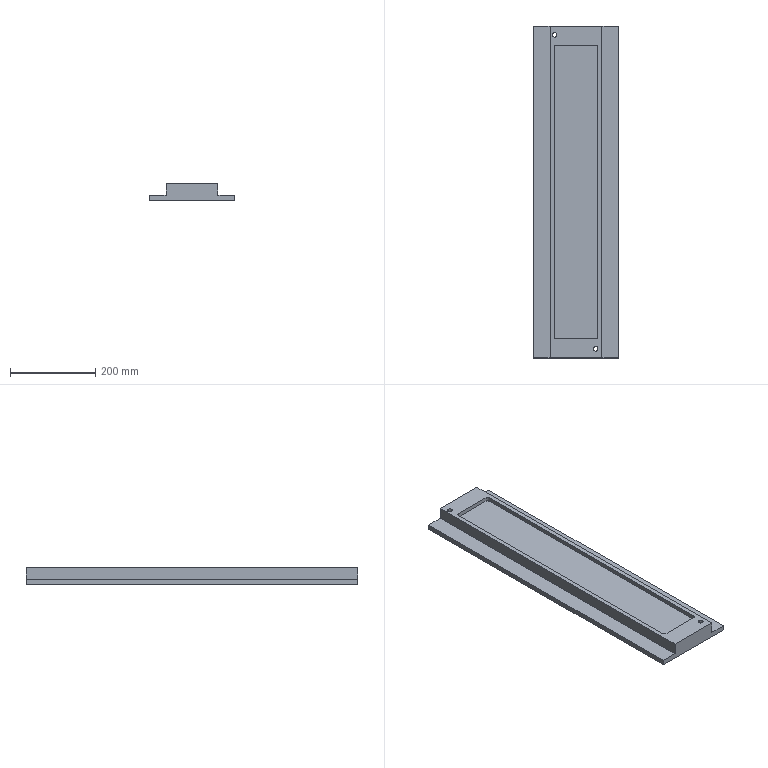Component | SolidWorks | Part43-1 | 1 solid | 23 faces | box 200 x 780 x 40 mm | volume 3825292 mm3 | plane 15 | cylinder 8 | commonest cylinder face diameters 11 x4 10 x4
build123d program:
from build123d import *

# Parameters (mm, degrees)
BOSS_EXTRUDE1_DEPTH = 390
CUT_EXTRUDE1_DEPTH  = 10
SKETCH3_R           = 5.5
CUT_EXTRUDE2_DEPTH  = 405.599


with BuildPart() as part:
    # Sketch1 → Boss-Extrude1 (new, symmetric)
    with BuildSketch(Plane(origin=(0, 0, 0), x_dir=(0, 0, -1), z_dir=(1, 0, 0))):
        Polygon((0, 100), (-12, 100), (-12, 61), (-40, 61), (-40, -61), (-12, -61), (-12, -100), (0, -100), align=None)
    extrude(amount=BOSS_EXTRUDE1_DEPTH, both=True)

    # Sketch2 → Cut-Extrude1 (cut)
    with BuildSketch(Plane.XY.offset(40)):
        with BuildLine():
            Line((-340, 51), (340, 51))
            ThreePointArc((340, 51), (343.536, 49.536), (345, 46))
            Line((345, 46), (345, -46))
            ThreePointArc((345, -46), (343.536, -49.536), (340, -51))
            Line((340, -51), (-340, -51))
            ThreePointArc((-340, -51), (-343.536, -49.536), (-345, -46))
            Line((-345, -46), (-345, 46))
            ThreePointArc((-345, 46), (-343.536, 49.536), (-340, 51))
        make_face()
    extrude(amount=-CUT_EXTRUDE1_DEPTH, mode=Mode.SUBTRACT)

    # Sketch3 → Cut-Extrude2 (cut, through all)
    with BuildSketch(Plane.XY.offset(40)):
        with Locations((-369.3, -50.2)):
            Circle(SKETCH3_R)
        with Locations((368.3, 46)):
            Circle(SKETCH3_R)
    extrude(amount=-CUT_EXTRUDE2_DEPTH, mode=Mode.SUBTRACT)


solid = part.part

# Placed as in the assembly
solid = solid.moved(Location((-87.007, -16, -360), (0, 0, -90)))
STEP:
#1=COLOUR_RGB('',0.7922,0.8196,0.9333);
#2=FILL_AREA_STYLE_COLOUR('',#1);
#3=FILL_AREA_STYLE('',(#2));
#4=SURFACE_STYLE_FILL_AREA(#3);
#5=SURFACE_SIDE_STYLE('',(#4));
#6=SURFACE_STYLE_USAGE(.BOTH.,#5);
#7=PRESENTATION_STYLE_ASSIGNMENT((#6));
#8=CARTESIAN_POINT('',(-1.614,-14.913,-14.173));
#9=VERTEX_POINT('',#8);
#10=CARTESIAN_POINT('',(-1.614,-15.346,-14.173));
#11=VERTEX_POINT('',#10);
#12=CARTESIAN_POINT('',(-1.614,-15.13,-14.173));
#13=DIRECTION('',(0.,0.,1.));
#14=DIRECTION('',(0.,-1.,0.));
#15=AXIS2_PLACEMENT_3D('',#12,#13,#14);
#16=CIRCLE('',#15,0.2165);
#17=EDGE_CURVE('',#9,#11,#16,.T.);
#18=ORIENTED_EDGE('',*,*,#17,.F.);
#19=CARTESIAN_POINT('',(-1.614,-14.913,-12.598));
#20=VERTEX_POINT('',#19);
#21=CARTESIAN_POINT('',(-1.614,-14.913,-14.173));
#22=DIRECTION('',(0.,0.,1.));
#23=VECTOR('',#22,39.37);
#24=LINE('',#21,#23);
#25=EDGE_CURVE('',#9,#20,#24,.T.);
#26=ORIENTED_EDGE('',*,*,#25,.T.);
#27=CARTESIAN_POINT('',(-1.614,-15.346,-12.598));
#28=VERTEX_POINT('',#27);
#29=CARTESIAN_POINT('',(-1.614,-15.13,-12.598));
#30=DIRECTION('',(0.,0.,1.));
#31=DIRECTION('',(0.,-1.,0.));
#32=AXIS2_PLACEMENT_3D('',#29,#30,#31);
#33=CIRCLE('',#32,0.2165);
#34=EDGE_CURVE('',#20,#28,#33,.T.);
#35=ORIENTED_EDGE('',*,*,#34,.T.);
#36=CARTESIAN_POINT('',(-1.614,-15.346,-14.173));
#37=DIRECTION('',(0.,0.,1.));
#38=VECTOR('',#37,39.37);
#39=LINE('',#36,#38);
#40=EDGE_CURVE('',#11,#28,#39,.T.);
#41=ORIENTED_EDGE('',*,*,#40,.F.);
#42=EDGE_LOOP('',(#18,#26,#35,#41));
#43=FACE_OUTER_BOUND('',#42,.T.);
#44=CARTESIAN_POINT('',(-1.614,-15.13,-14.173));
#45=DIRECTION('',(0.,0.,1.));
#46=DIRECTION('',(0.,-1.,0.));
#47=AXIS2_PLACEMENT_3D('',#44,#45,#46);
#48=CYLINDRICAL_SURFACE('',#47,0.2165);
#49=ADVANCED_FACE('',(#43),#48,.F.);
#50=CARTESIAN_POINT('',(-5.402,14.126,-14.173));
#51=VERTEX_POINT('',#50);
#52=CARTESIAN_POINT('',(-5.402,13.693,-14.173));
#53=VERTEX_POINT('',#52);
#54=CARTESIAN_POINT('',(-5.402,13.909,-14.173));
#55=DIRECTION('',(0.,0.,1.));
#56=DIRECTION('',(0.,-1.,0.));
#57=AXIS2_PLACEMENT_3D('',#54,#55,#56);
#58=CIRCLE('',#57,0.2165);
#59=EDGE_CURVE('',#51,#53,#58,.T.);
#60=ORIENTED_EDGE('',*,*,#59,.F.);
#61=CARTESIAN_POINT('',(-5.402,14.126,-12.598));
#62=VERTEX_POINT('',#61);
#63=CARTESIAN_POINT('',(-5.402,14.126,-14.173));
#64=DIRECTION('',(0.,0.,1.));
#65=VECTOR('',#64,39.37);
#66=LINE('',#63,#65);
#67=EDGE_CURVE('',#51,#62,#66,.T.);
#68=ORIENTED_EDGE('',*,*,#67,.T.);
#69=CARTESIAN_POINT('',(-5.402,13.693,-12.598));
#70=VERTEX_POINT('',#69);
#71=CARTESIAN_POINT('',(-5.402,13.909,-12.598));
#72=DIRECTION('',(0.,0.,1.));
#73=DIRECTION('',(0.,-1.,0.));
#74=AXIS2_PLACEMENT_3D('',#71,#72,#73);
#75=CIRCLE('',#74,0.2165);
#76=EDGE_CURVE('',#62,#70,#75,.T.);
#77=ORIENTED_EDGE('',*,*,#76,.T.);
#78=CARTESIAN_POINT('',(-5.402,13.693,-14.173));
#79=DIRECTION('',(0.,0.,1.));
#80=VECTOR('',#79,39.37);
#81=LINE('',#78,#80);
#82=EDGE_CURVE('',#53,#70,#81,.T.);
#83=ORIENTED_EDGE('',*,*,#82,.F.);
#84=EDGE_LOOP('',(#60,#68,#77,#83));
#85=FACE_OUTER_BOUND('',#84,.T.);
#86=CARTESIAN_POINT('',(-5.402,13.909,-14.173));
#87=DIRECTION('',(0.,0.,1.));
#88=DIRECTION('',(0.,-1.,0.));
#89=AXIS2_PLACEMENT_3D('',#86,#87,#88);
#90=CYLINDRICAL_SURFACE('',#89,0.2165);
#91=ADVANCED_FACE('',(#85),#90,.F.);
#92=CARTESIAN_POINT('',(-1.614,-15.13,-14.173));
#93=DIRECTION('',(0.,0.,1.));
#94=DIRECTION('',(0.,-1.,0.));
#95=AXIS2_PLACEMENT_3D('',#92,#93,#94);
#96=CIRCLE('',#95,0.2165);
#97=EDGE_CURVE('',#11,#9,#96,.T.);
#98=ORIENTED_EDGE('',*,*,#97,.T.);
#99=ORIENTED_EDGE('',*,*,#17,.T.);
#100=EDGE_LOOP('',(#98,#99));
#101=FACE_BOUND('',#100,.T.);
#102=CARTESIAN_POINT('',(-5.402,13.909,-14.173));
#103=DIRECTION('',(0.,0.,1.));
#104=DIRECTION('',(0.,-1.,0.));
#105=AXIS2_PLACEMENT_3D('',#102,#103,#104);
#106=CIRCLE('',#105,0.2165);
#107=EDGE_CURVE('',#53,#51,#106,.T.);
#108=ORIENTED_EDGE('',*,*,#107,.T.);
#109=ORIENTED_EDGE('',*,*,#59,.T.);
#110=EDGE_LOOP('',(#108,#109));
#111=FACE_BOUND('',#110,.T.);
#112=CARTESIAN_POINT('',(-7.362,14.724,-14.173));
#113=VERTEX_POINT('',#112);
#114=CARTESIAN_POINT('',(0.5115,14.724,-14.173));
#115=VERTEX_POINT('',#114);
#116=CARTESIAN_POINT('',(0.5115,14.724,-14.173));
#117=DIRECTION('',(1.,0.,-0.));
#118=VECTOR('',#117,39.37);
#119=LINE('',#116,#118);
#120=EDGE_CURVE('',#113,#115,#119,.T.);
#121=ORIENTED_EDGE('',*,*,#120,.T.);
#122=CARTESIAN_POINT('',(0.5115,-15.984,-14.173));
#123=VERTEX_POINT('',#122);
#124=CARTESIAN_POINT('',(0.5115,-15.984,-14.173));
#125=DIRECTION('',(-0.,1.,-0.));
#126=VECTOR('',#125,39.37);
#127=LINE('',#124,#126);
#128=EDGE_CURVE('',#123,#115,#127,.T.);
#129=ORIENTED_EDGE('',*,*,#128,.F.);
#130=CARTESIAN_POINT('',(-7.362,-15.984,-14.173));
#131=VERTEX_POINT('',#130);
#132=CARTESIAN_POINT('',(0.5115,-15.984,-14.173));
#133=DIRECTION('',(1.,0.,-0.));
#134=VECTOR('',#133,39.37);
#135=LINE('',#132,#134);
#136=EDGE_CURVE('',#131,#123,#135,.T.);
#137=ORIENTED_EDGE('',*,*,#136,.F.);
#138=CARTESIAN_POINT('',(-7.362,-15.984,-14.173));
#139=DIRECTION('',(-0.,1.,-0.));
#140=VECTOR('',#139,39.37);
#141=LINE('',#138,#140);
#142=EDGE_CURVE('',#131,#113,#141,.T.);
#143=ORIENTED_EDGE('',*,*,#142,.T.);
#144=EDGE_LOOP('',(#121,#129,#137,#143));
#145=FACE_OUTER_BOUND('',#144,.T.);
#146=CARTESIAN_POINT('',(0.5115,-15.984,-14.173));
#147=DIRECTION('',(0.,0.,1.));
#148=DIRECTION('',(-1.,-0.,0.));
#149=AXIS2_PLACEMENT_3D('',#146,#147,#148);
#150=PLANE('',#149);
#151=ADVANCED_FACE('',(#101,#111,#145),#150,.F.);
#152=CARTESIAN_POINT('',(0.5115,14.724,-13.701));
#153=VERTEX_POINT('',#152);
#154=CARTESIAN_POINT('',(0.5115,14.724,-14.173));
#155=DIRECTION('',(0.,0.,1.));
#156=VECTOR('',#155,39.37);
#157=LINE('',#154,#156);
#158=EDGE_CURVE('',#115,#153,#157,.T.);
#159=ORIENTED_EDGE('',*,*,#158,.T.);
#160=CARTESIAN_POINT('',(0.5115,-15.984,-13.701));
#161=VERTEX_POINT('',#160);
#162=CARTESIAN_POINT('',(0.5115,-15.984,-13.701));
#163=DIRECTION('',(-0.,1.,-0.));
#164=VECTOR('',#163,39.37);
#165=LINE('',#162,#164);
#166=EDGE_CURVE('',#161,#153,#165,.T.);
#167=ORIENTED_EDGE('',*,*,#166,.F.);
#168=CARTESIAN_POINT('',(0.5115,-15.984,-14.173));
#169=DIRECTION('',(0.,0.,1.));
#170=VECTOR('',#169,39.37);
#171=LINE('',#168,#170);
#172=EDGE_CURVE('',#123,#161,#171,.T.);
#173=ORIENTED_EDGE('',*,*,#172,.F.);
#174=ORIENTED_EDGE('',*,*,#128,.T.);
#175=EDGE_LOOP('',(#159,#167,#173,#174));
#176=FACE_OUTER_BOUND('',#175,.T.);
#177=CARTESIAN_POINT('',(0.5115,-15.984,-14.173));
#178=DIRECTION('',(-1.,-0.,0.));
#179=DIRECTION('',(-0.,-0.,-1.));
#180=AXIS2_PLACEMENT_3D('',#177,#178,#179);
#181=PLANE('',#180);
#182=ADVANCED_FACE('',(#176),#181,.F.);
#183=CARTESIAN_POINT('',(-1.024,14.724,-13.701));
#184=VERTEX_POINT('',#183);
#185=CARTESIAN_POINT('',(0.5115,14.724,-13.701));
#186=DIRECTION('',(-1.,-0.,0.));
#187=VECTOR('',#186,39.37);
#188=LINE('',#185,#187);
#189=EDGE_CURVE('',#153,#184,#188,.T.);
#190=ORIENTED_EDGE('',*,*,#189,.T.);
#191=CARTESIAN_POINT('',(-1.024,-15.984,-13.701));
#192=VERTEX_POINT('',#191);
#193=CARTESIAN_POINT('',(-1.024,-15.984,-13.701));
#194=DIRECTION('',(-0.,1.,-0.));
#195=VECTOR('',#194,39.37);
#196=LINE('',#193,#195);
#197=EDGE_CURVE('',#192,#184,#196,.T.);
#198=ORIENTED_EDGE('',*,*,#197,.F.);
#199=CARTESIAN_POINT('',(0.5115,-15.984,-13.701));
#200=DIRECTION('',(-1.,-0.,0.));
#201=VECTOR('',#200,39.37);
#202=LINE('',#199,#201);
#203=EDGE_CURVE('',#161,#192,#202,.T.);
#204=ORIENTED_EDGE('',*,*,#203,.F.);
#205=ORIENTED_EDGE('',*,*,#166,.T.);
#206=EDGE_LOOP('',(#190,#198,#204,#205));
#207=FACE_OUTER_BOUND('',#206,.T.);
#208=CARTESIAN_POINT('',(0.5115,-15.984,-13.701));
#209=DIRECTION('',(-0.,-0.,-1.));
#210=DIRECTION('',(1.,0.,-0.));
#211=AXIS2_PLACEMENT_3D('',#208,#209,#210);
#212=PLANE('',#211);
#213=ADVANCED_FACE('',(#207),#212,.F.);
#214=CARTESIAN_POINT('',(-1.024,14.724,-12.598));
#215=VERTEX_POINT('',#214);
#216=CARTESIAN_POINT('',(-1.024,14.724,-13.701));
#217=DIRECTION('',(0.,0.,1.));
#218=VECTOR('',#217,39.37);
#219=LINE('',#216,#218);
#220=EDGE_CURVE('',#184,#215,#219,.T.);
#221=ORIENTED_EDGE('',*,*,#220,.T.);
#222=CARTESIAN_POINT('',(-1.024,-15.984,-12.598));
#223=VERTEX_POINT('',#222);
#224=CARTESIAN_POINT('',(-1.024,-15.984,-12.598));
#225=DIRECTION('',(-0.,1.,-0.));
#226=VECTOR('',#225,39.37);
#227=LINE('',#224,#226);
#228=EDGE_CURVE('',#223,#215,#227,.T.);
#229=ORIENTED_EDGE('',*,*,#228,.F.);
#230=CARTESIAN_POINT('',(-1.024,-15.984,-13.701));
#231=DIRECTION('',(0.,0.,1.));
#232=VECTOR('',#231,39.37);
#233=LINE('',#230,#232);
#234=EDGE_CURVE('',#192,#223,#233,.T.);
#235=ORIENTED_EDGE('',*,*,#234,.F.);
#236=ORIENTED_EDGE('',*,*,#197,.T.);
#237=EDGE_LOOP('',(#221,#229,#235,#236));
#238=FACE_OUTER_BOUND('',#237,.T.);
#239=CARTESIAN_POINT('',(-1.024,-15.984,-13.701));
#240=DIRECTION('',(-1.,-0.,0.));
#241=DIRECTION('',(-0.,-0.,-1.));
#242=AXIS2_PLACEMENT_3D('',#239,#240,#241);
#243=PLANE('',#242);
#244=ADVANCED_FACE('',(#238),#243,.F.);
#245=CARTESIAN_POINT('',(-1.614,-15.13,-12.598));
#246=DIRECTION('',(0.,0.,1.));
#247=DIRECTION('',(0.,-1.,0.));
#248=AXIS2_PLACEMENT_3D('',#245,#246,#247);
#249=CIRCLE('',#248,0.2165);
#250=EDGE_CURVE('',#28,#20,#249,.T.);
#251=ORIENTED_EDGE('',*,*,#250,.F.);
#252=ORIENTED_EDGE('',*,*,#34,.F.);
#253=EDGE_LOOP('',(#251,#252));
#254=FACE_BOUND('',#253,.T.);
#255=CARTESIAN_POINT('',(-5.402,13.909,-12.598));
#256=DIRECTION('',(0.,0.,1.));
#257=DIRECTION('',(0.,-1.,0.));
#258=AXIS2_PLACEMENT_3D('',#255,#256,#257);
#259=CIRCLE('',#258,0.2165);
#260=EDGE_CURVE('',#70,#62,#259,.T.);
#261=ORIENTED_EDGE('',*,*,#260,.F.);
#262=ORIENTED_EDGE('',*,*,#76,.F.);
#263=EDGE_LOOP('',(#261,#262));
#264=FACE_BOUND('',#263,.T.);
#265=CARTESIAN_POINT('',(-1.418,-14.016,-12.598));
#266=VERTEX_POINT('',#265);
#267=CARTESIAN_POINT('',(-1.418,12.756,-12.598));
#268=VERTEX_POINT('',#267);
#269=CARTESIAN_POINT('',(-1.418,12.756,-12.598));
#270=DIRECTION('',(-0.,1.,-0.));
#271=VECTOR('',#270,39.37);
#272=LINE('',#269,#271);
#273=EDGE_CURVE('',#266,#268,#272,.T.);
#274=ORIENTED_EDGE('',*,*,#273,.F.);
#275=CARTESIAN_POINT('',(-1.614,-14.213,-12.598));
#276=VERTEX_POINT('',#275);
#277=CARTESIAN_POINT('',(-1.614,-14.016,-12.598));
#278=DIRECTION('',(0.,0.,1.));
#279=DIRECTION('',(0.,1.,0.));
#280=AXIS2_PLACEMENT_3D('',#277,#278,#279);
#281=CIRCLE('',#280,0.1969);
#282=EDGE_CURVE('',#276,#266,#281,.T.);
#283=ORIENTED_EDGE('',*,*,#282,.F.);
#284=CARTESIAN_POINT('',(-5.236,-14.213,-12.598));
#285=VERTEX_POINT('',#284);
#286=CARTESIAN_POINT('',(-1.614,-14.213,-12.598));
#287=DIRECTION('',(1.,0.,-0.));
#288=VECTOR('',#287,39.37);
#289=LINE('',#286,#288);
#290=EDGE_CURVE('',#285,#276,#289,.T.);
#291=ORIENTED_EDGE('',*,*,#290,.F.);
#292=CARTESIAN_POINT('',(-5.433,-14.016,-12.598));
#293=VERTEX_POINT('',#292);
#294=CARTESIAN_POINT('',(-5.236,-14.016,-12.598));
#295=DIRECTION('',(0.,0.,1.));
#296=DIRECTION('',(0.,-1.,0.));
#297=AXIS2_PLACEMENT_3D('',#294,#295,#296);
#298=CIRCLE('',#297,0.1969);
#299=EDGE_CURVE('',#293,#285,#298,.T.);
#300=ORIENTED_EDGE('',*,*,#299,.F.);
#301=CARTESIAN_POINT('',(-5.433,12.756,-12.598));
#302=VERTEX_POINT('',#301);
#303=CARTESIAN_POINT('',(-5.433,12.756,-12.598));
#304=DIRECTION('',(0.,-1.,0.));
#305=VECTOR('',#304,39.37);
#306=LINE('',#303,#305);
#307=EDGE_CURVE('',#302,#293,#306,.T.);
#308=ORIENTED_EDGE('',*,*,#307,.F.);
#309=CARTESIAN_POINT('',(-5.236,12.953,-12.598));
#310=VERTEX_POINT('',#309);
#311=CARTESIAN_POINT('',(-5.236,12.756,-12.598));
#312=DIRECTION('',(0.,0.,1.));
#313=DIRECTION('',(0.,-1.,0.));
#314=AXIS2_PLACEMENT_3D('',#311,#312,#313);
#315=CIRCLE('',#314,0.1969);
#316=EDGE_CURVE('',#310,#302,#315,.T.);
#317=ORIENTED_EDGE('',*,*,#316,.F.);
#318=CARTESIAN_POINT('',(-1.614,12.953,-12.598));
#319=VERTEX_POINT('',#318);
#320=CARTESIAN_POINT('',(-1.614,12.953,-12.598));
#321=DIRECTION('',(-1.,0.,0.));
#322=VECTOR('',#321,39.37);
#323=LINE('',#320,#322);
#324=EDGE_CURVE('',#319,#310,#323,.T.);
#325=ORIENTED_EDGE('',*,*,#324,.F.);
#326=CARTESIAN_POINT('',(-1.614,12.756,-12.598));
#327=DIRECTION('',(0.,0.,1.));
#328=DIRECTION('',(0.,-1.,0.));
#329=AXIS2_PLACEMENT_3D('',#326,#327,#328);
#330=CIRCLE('',#329,0.1969);
#331=EDGE_CURVE('',#268,#319,#330,.T.);
#332=ORIENTED_EDGE('',*,*,#331,.F.);
#333=EDGE_LOOP('',(#274,#283,#291,#300,#308,#317,#325,#332));
#334=FACE_BOUND('',#333,.T.);
#335=CARTESIAN_POINT('',(-5.827,14.724,-12.598));
#336=VERTEX_POINT('',#335);
#337=CARTESIAN_POINT('',(-1.024,14.724,-12.598));
#338=DIRECTION('',(-1.,-0.,0.));
#339=VECTOR('',#338,39.37);
#340=LINE('',#337,#339);
#341=EDGE_CURVE('',#215,#336,#340,.T.);
#342=ORIENTED_EDGE('',*,*,#341,.T.);
#343=CARTESIAN_POINT('',(-5.827,-15.984,-12.598));
#344=VERTEX_POINT('',#343);
#345=CARTESIAN_POINT('',(-5.827,-15.984,-12.598));
#346=DIRECTION('',(-0.,1.,-0.));
#347=VECTOR('',#346,39.37);
#348=LINE('',#345,#347);
#349=EDGE_CURVE('',#344,#336,#348,.T.);
#350=ORIENTED_EDGE('',*,*,#349,.F.);
#351=CARTESIAN_POINT('',(-1.024,-15.984,-12.598));
#352=DIRECTION('',(-1.,-0.,0.));
#353=VECTOR('',#352,39.37);
#354=LINE('',#351,#353);
#355=EDGE_CURVE('',#223,#344,#354,.T.);
#356=ORIENTED_EDGE('',*,*,#355,.F.);
#357=ORIENTED_EDGE('',*,*,#228,.T.);
#358=EDGE_LOOP('',(#342,#350,#356,#357));
#359=FACE_OUTER_BOUND('',#358,.T.);
#360=CARTESIAN_POINT('',(-1.024,-15.984,-12.598));
#361=DIRECTION('',(-0.,-0.,-1.));
#362=DIRECTION('',(1.,0.,-0.));
#363=AXIS2_PLACEMENT_3D('',#360,#361,#362);
#364=PLANE('',#363);
#365=ADVANCED_FACE('',(#254,#264,#334,#359),#364,.F.);
#366=CARTESIAN_POINT('',(-5.827,14.724,-13.701));
#367=VERTEX_POINT('',#366);
#368=CARTESIAN_POINT('',(-5.827,14.724,-13.701));
#369=DIRECTION('',(-0.,-0.,-1.));
#370=VECTOR('',#369,39.37);
#371=LINE('',#368,#370);
#372=EDGE_CURVE('',#336,#367,#371,.T.);
#373=ORIENTED_EDGE('',*,*,#372,.T.);
#374=CARTESIAN_POINT('',(-5.827,-15.984,-13.701));
#375=VERTEX_POINT('',#374);
#376=CARTESIAN_POINT('',(-5.827,-15.984,-13.701));
#377=DIRECTION('',(-0.,1.,-0.));
#378=VECTOR('',#377,39.37);
#379=LINE('',#376,#378);
#380=EDGE_CURVE('',#375,#367,#379,.T.);
#381=ORIENTED_EDGE('',*,*,#380,.F.);
#382=CARTESIAN_POINT('',(-5.827,-15.984,-13.701));
#383=DIRECTION('',(-0.,-0.,-1.));
#384=VECTOR('',#383,39.37);
#385=LINE('',#382,#384);
#386=EDGE_CURVE('',#344,#375,#385,.T.);
#387=ORIENTED_EDGE('',*,*,#386,.F.);
#388=ORIENTED_EDGE('',*,*,#349,.T.);
#389=EDGE_LOOP('',(#373,#381,#387,#388));
#390=FACE_OUTER_BOUND('',#389,.T.);
#391=CARTESIAN_POINT('',(-5.827,-15.984,-13.701));
#392=DIRECTION('',(1.,0.,-0.));
#393=DIRECTION('',(0.,0.,1.));
#394=AXIS2_PLACEMENT_3D('',#391,#392,#393);
#395=PLANE('',#394);
#396=ADVANCED_FACE('',(#390),#395,.F.);
#397=CARTESIAN_POINT('',(-7.362,14.724,-13.701));
#398=VERTEX_POINT('',#397);
#399=CARTESIAN_POINT('',(-5.827,14.724,-13.701));
#400=DIRECTION('',(-1.,-0.,0.));
#401=VECTOR('',#400,39.37);
#402=LINE('',#399,#401);
#403=EDGE_CURVE('',#367,#398,#402,.T.);
#404=ORIENTED_EDGE('',*,*,#403,.T.);
#405=CARTESIAN_POINT('',(-7.362,-15.984,-13.701));
#406=VERTEX_POINT('',#405);
#407=CARTESIAN_POINT('',(-7.362,-15.984,-13.701));
#408=DIRECTION('',(-0.,1.,-0.));
#409=VECTOR('',#408,39.37);
#410=LINE('',#407,#409);
#411=EDGE_CURVE('',#406,#398,#410,.T.);
#412=ORIENTED_EDGE('',*,*,#411,.F.);
#413=CARTESIAN_POINT('',(-5.827,-15.984,-13.701));
#414=DIRECTION('',(-1.,-0.,0.));
#415=VECTOR('',#414,39.37);
#416=LINE('',#413,#415);
#417=EDGE_CURVE('',#375,#406,#416,.T.);
#418=ORIENTED_EDGE('',*,*,#417,.F.);
#419=ORIENTED_EDGE('',*,*,#380,.T.);
#420=EDGE_LOOP('',(#404,#412,#418,#419));
#421=FACE_OUTER_BOUND('',#420,.T.);
#422=CARTESIAN_POINT('',(-5.827,-15.984,-13.701));
#423=DIRECTION('',(-0.,-0.,-1.));
#424=DIRECTION('',(1.,0.,-0.));
#425=AXIS2_PLACEMENT_3D('',#422,#423,#424);
#426=PLANE('',#425);
#427=ADVANCED_FACE('',(#421),#426,.F.);
#428=CARTESIAN_POINT('',(-7.362,14.724,-14.173));
#429=DIRECTION('',(-0.,-0.,-1.));
#430=VECTOR('',#429,39.37);
#431=LINE('',#428,#430);
#432=EDGE_CURVE('',#398,#113,#431,.T.);
#433=ORIENTED_EDGE('',*,*,#432,.T.);
#434=ORIENTED_EDGE('',*,*,#142,.F.);
#435=CARTESIAN_POINT('',(-7.362,-15.984,-14.173));
#436=DIRECTION('',(-0.,-0.,-1.));
#437=VECTOR('',#436,39.37);
#438=LINE('',#435,#437);
#439=EDGE_CURVE('',#406,#131,#438,.T.);
#440=ORIENTED_EDGE('',*,*,#439,.F.);
#441=ORIENTED_EDGE('',*,*,#411,.T.);
#442=EDGE_LOOP('',(#433,#434,#440,#441));
#443=FACE_OUTER_BOUND('',#442,.T.);
#444=CARTESIAN_POINT('',(-7.362,-15.984,-14.173));
#445=DIRECTION('',(1.,0.,-0.));
#446=DIRECTION('',(0.,0.,1.));
#447=AXIS2_PLACEMENT_3D('',#444,#445,#446);
#448=PLANE('',#447);
#449=ADVANCED_FACE('',(#443),#448,.F.);
#450=ORIENTED_EDGE('',*,*,#136,.T.);
#451=ORIENTED_EDGE('',*,*,#172,.T.);
#452=ORIENTED_EDGE('',*,*,#203,.T.);
#453=ORIENTED_EDGE('',*,*,#234,.T.);
#454=ORIENTED_EDGE('',*,*,#355,.T.);
#455=ORIENTED_EDGE('',*,*,#386,.T.);
#456=ORIENTED_EDGE('',*,*,#417,.T.);
#457=ORIENTED_EDGE('',*,*,#439,.T.);
#458=EDGE_LOOP('',(#450,#451,#452,#453,#454,#455,#456,#457));
#459=FACE_OUTER_BOUND('',#458,.T.);
#460=CARTESIAN_POINT('',(-3.425,-15.984,-14.173));
#461=DIRECTION('',(-0.,1.,-0.));
#462=DIRECTION('',(0.,0.,1.));
#463=AXIS2_PLACEMENT_3D('',#460,#461,#462);
#464=PLANE('',#463);
#465=ADVANCED_FACE('',(#459),#464,.F.);
#466=ORIENTED_EDGE('',*,*,#120,.F.);
#467=ORIENTED_EDGE('',*,*,#432,.F.);
#468=ORIENTED_EDGE('',*,*,#403,.F.);
#469=ORIENTED_EDGE('',*,*,#372,.F.);
#470=ORIENTED_EDGE('',*,*,#341,.F.);
#471=ORIENTED_EDGE('',*,*,#220,.F.);
#472=ORIENTED_EDGE('',*,*,#189,.F.);
#473=ORIENTED_EDGE('',*,*,#158,.F.);
#474=EDGE_LOOP('',(#466,#467,#468,#469,#470,#471,#472,#473));
#475=FACE_OUTER_BOUND('',#474,.T.);
#476=CARTESIAN_POINT('',(-3.425,14.724,-14.173));
#477=DIRECTION('',(-0.,1.,-0.));
#478=DIRECTION('',(0.,0.,1.));
#479=AXIS2_PLACEMENT_3D('',#476,#477,#478);
#480=PLANE('',#479);
#481=ADVANCED_FACE('',(#475),#480,.T.);
#482=ORIENTED_EDGE('',*,*,#282,.T.);
#483=CARTESIAN_POINT('',(-1.418,-14.016,-12.992));
#484=VERTEX_POINT('',#483);
#485=CARTESIAN_POINT('',(-1.418,-14.016,-12.992));
#486=DIRECTION('',(0.,0.,1.));
#487=VECTOR('',#486,39.37);
#488=LINE('',#485,#487);
#489=EDGE_CURVE('',#484,#266,#488,.T.);
#490=ORIENTED_EDGE('',*,*,#489,.F.);
#491=CARTESIAN_POINT('',(-1.614,-14.213,-12.992));
#492=VERTEX_POINT('',#491);
#493=CARTESIAN_POINT('',(-1.614,-14.016,-12.992));
#494=DIRECTION('',(0.,0.,1.));
#495=DIRECTION('',(0.,1.,0.));
#496=AXIS2_PLACEMENT_3D('',#493,#494,#495);
#497=CIRCLE('',#496,0.1969);
#498=EDGE_CURVE('',#492,#484,#497,.T.);
#499=ORIENTED_EDGE('',*,*,#498,.F.);
#500=CARTESIAN_POINT('',(-1.614,-14.213,-12.992));
#501=DIRECTION('',(0.,0.,1.));
#502=VECTOR('',#501,39.37);
#503=LINE('',#500,#502);
#504=EDGE_CURVE('',#492,#276,#503,.T.);
#505=ORIENTED_EDGE('',*,*,#504,.T.);
#506=EDGE_LOOP('',(#482,#490,#499,#505));
#507=FACE_OUTER_BOUND('',#506,.T.);
#508=CARTESIAN_POINT('',(-1.614,-14.016,-12.992));
#509=DIRECTION('',(0.,0.,1.));
#510=DIRECTION('',(0.,-1.,0.));
#511=AXIS2_PLACEMENT_3D('',#508,#509,#510);
#512=CYLINDRICAL_SURFACE('',#511,0.1969);
#513=ADVANCED_FACE('',(#507),#512,.F.);
#514=ORIENTED_EDGE('',*,*,#290,.T.);
#515=ORIENTED_EDGE('',*,*,#504,.F.);
#516=CARTESIAN_POINT('',(-5.236,-14.213,-12.992));
#517=VERTEX_POINT('',#516);
#518=CARTESIAN_POINT('',(-1.614,-14.213,-12.992));
#519=DIRECTION('',(1.,0.,-0.));
#520=VECTOR('',#519,39.37);
#521=LINE('',#518,#520);
#522=EDGE_CURVE('',#517,#492,#521,.T.);
#523=ORIENTED_EDGE('',*,*,#522,.F.);
#524=CARTESIAN_POINT('',(-5.236,-14.213,-12.992));
#525=DIRECTION('',(0.,0.,1.));
#526=VECTOR('',#525,39.37);
#527=LINE('',#524,#526);
#528=EDGE_CURVE('',#517,#285,#527,.T.);
#529=ORIENTED_EDGE('',*,*,#528,.T.);
#530=EDGE_LOOP('',(#514,#515,#523,#529));
#531=FACE_OUTER_BOUND('',#530,.T.);
#532=CARTESIAN_POINT('',(-1.614,-14.213,-12.992));
#533=DIRECTION('',(0.,-1.,0.));
#534=DIRECTION('',(-0.,-0.,-1.));
#535=AXIS2_PLACEMENT_3D('',#532,#533,#534);
#536=PLANE('',#535);
#537=ADVANCED_FACE('',(#531),#536,.F.);
#538=ORIENTED_EDGE('',*,*,#299,.T.);
#539=ORIENTED_EDGE('',*,*,#528,.F.);
#540=CARTESIAN_POINT('',(-5.433,-14.016,-12.992));
#541=VERTEX_POINT('',#540);
#542=CARTESIAN_POINT('',(-5.236,-14.016,-12.992));
#543=DIRECTION('',(0.,0.,1.));
#544=DIRECTION('',(0.,-1.,0.));
#545=AXIS2_PLACEMENT_3D('',#542,#543,#544);
#546=CIRCLE('',#545,0.1969);
#547=EDGE_CURVE('',#541,#517,#546,.T.);
#548=ORIENTED_EDGE('',*,*,#547,.F.);
#549=CARTESIAN_POINT('',(-5.433,-14.016,-12.992));
#550=DIRECTION('',(0.,0.,1.));
#551=VECTOR('',#550,39.37);
#552=LINE('',#549,#551);
#553=EDGE_CURVE('',#541,#293,#552,.T.);
#554=ORIENTED_EDGE('',*,*,#553,.T.);
#555=EDGE_LOOP('',(#538,#539,#548,#554));
#556=FACE_OUTER_BOUND('',#555,.T.);
#557=CARTESIAN_POINT('',(-5.236,-14.016,-12.992));
#558=DIRECTION('',(0.,0.,1.));
#559=DIRECTION('',(0.,-1.,0.));
#560=AXIS2_PLACEMENT_3D('',#557,#558,#559);
#561=CYLINDRICAL_SURFACE('',#560,0.1969);
#562=ADVANCED_FACE('',(#556),#561,.F.);
#563=ORIENTED_EDGE('',*,*,#307,.T.);
#564=ORIENTED_EDGE('',*,*,#553,.F.);
#565=CARTESIAN_POINT('',(-5.433,12.756,-12.992));
#566=VERTEX_POINT('',#565);
#567=CARTESIAN_POINT('',(-5.433,12.756,-12.992));
#568=DIRECTION('',(0.,-1.,0.));
#569=VECTOR('',#568,39.37);
#570=LINE('',#567,#569);
#571=EDGE_CURVE('',#566,#541,#570,.T.);
#572=ORIENTED_EDGE('',*,*,#571,.F.);
#573=CARTESIAN_POINT('',(-5.433,12.756,-12.992));
#574=DIRECTION('',(0.,0.,1.));
#575=VECTOR('',#574,39.37);
#576=LINE('',#573,#575);
#577=EDGE_CURVE('',#566,#302,#576,.T.);
#578=ORIENTED_EDGE('',*,*,#577,.T.);
#579=EDGE_LOOP('',(#563,#564,#572,#578));
#580=FACE_OUTER_BOUND('',#579,.T.);
#581=CARTESIAN_POINT('',(-5.433,12.756,-12.992));
#582=DIRECTION('',(-1.,-0.,0.));
#583=DIRECTION('',(-0.,-0.,-1.));
#584=AXIS2_PLACEMENT_3D('',#581,#582,#583);
#585=PLANE('',#584);
#586=ADVANCED_FACE('',(#580),#585,.F.);
#587=ORIENTED_EDGE('',*,*,#316,.T.);
#588=ORIENTED_EDGE('',*,*,#577,.F.);
#589=CARTESIAN_POINT('',(-5.236,12.953,-12.992));
#590=VERTEX_POINT('',#589);
#591=CARTESIAN_POINT('',(-5.236,12.756,-12.992));
#592=DIRECTION('',(0.,0.,1.));
#593=DIRECTION('',(0.,-1.,0.));
#594=AXIS2_PLACEMENT_3D('',#591,#592,#593);
#595=CIRCLE('',#594,0.1969);
#596=EDGE_CURVE('',#590,#566,#595,.T.);
#597=ORIENTED_EDGE('',*,*,#596,.F.);
#598=CARTESIAN_POINT('',(-5.236,12.953,-12.992));
#599=DIRECTION('',(0.,0.,1.));
#600=VECTOR('',#599,39.37);
#601=LINE('',#598,#600);
#602=EDGE_CURVE('',#590,#310,#601,.T.);
#603=ORIENTED_EDGE('',*,*,#602,.T.);
#604=EDGE_LOOP('',(#587,#588,#597,#603));
#605=FACE_OUTER_BOUND('',#604,.T.);
#606=CARTESIAN_POINT('',(-5.236,12.756,-12.992));
#607=DIRECTION('',(0.,0.,1.));
#608=DIRECTION('',(0.,-1.,0.));
#609=AXIS2_PLACEMENT_3D('',#606,#607,#608);
#610=CYLINDRICAL_SURFACE('',#609,0.1969);
#611=ADVANCED_FACE('',(#605),#610,.F.);
#612=ORIENTED_EDGE('',*,*,#324,.T.);
#613=ORIENTED_EDGE('',*,*,#602,.F.);
#614=CARTESIAN_POINT('',(-1.614,12.953,-12.992));
#615=VERTEX_POINT('',#614);
#616=CARTESIAN_POINT('',(-1.614,12.953,-12.992));
#617=DIRECTION('',(-1.,0.,0.));
#618=VECTOR('',#617,39.37);
#619=LINE('',#616,#618);
#620=EDGE_CURVE('',#615,#590,#619,.T.);
#621=ORIENTED_EDGE('',*,*,#620,.F.);
#622=CARTESIAN_POINT('',(-1.614,12.953,-12.992));
#623=DIRECTION('',(0.,0.,1.));
#624=VECTOR('',#623,39.37);
#625=LINE('',#622,#624);
#626=EDGE_CURVE('',#615,#319,#625,.T.);
#627=ORIENTED_EDGE('',*,*,#626,.T.);
#628=EDGE_LOOP('',(#612,#613,#621,#627));
#629=FACE_OUTER_BOUND('',#628,.T.);
#630=CARTESIAN_POINT('',(-1.614,12.953,-12.992));
#631=DIRECTION('',(0.,1.,-0.));
#632=DIRECTION('',(-1.,0.,0.));
#633=AXIS2_PLACEMENT_3D('',#630,#631,#632);
#634=PLANE('',#633);
#635=ADVANCED_FACE('',(#629),#634,.F.);
#636=ORIENTED_EDGE('',*,*,#331,.T.);
#637=ORIENTED_EDGE('',*,*,#626,.F.);
#638=CARTESIAN_POINT('',(-1.418,12.756,-12.992));
#639=VERTEX_POINT('',#638);
#640=CARTESIAN_POINT('',(-1.614,12.756,-12.992));
#641=DIRECTION('',(0.,0.,1.));
#642=DIRECTION('',(0.,-1.,0.));
#643=AXIS2_PLACEMENT_3D('',#640,#641,#642);
#644=CIRCLE('',#643,0.1969);
#645=EDGE_CURVE('',#639,#615,#644,.T.);
#646=ORIENTED_EDGE('',*,*,#645,.F.);
#647=CARTESIAN_POINT('',(-1.418,12.756,-12.992));
#648=DIRECTION('',(0.,0.,1.));
#649=VECTOR('',#648,39.37);
#650=LINE('',#647,#649);
#651=EDGE_CURVE('',#639,#268,#650,.T.);
#652=ORIENTED_EDGE('',*,*,#651,.T.);
#653=EDGE_LOOP('',(#636,#637,#646,#652));
#654=FACE_OUTER_BOUND('',#653,.T.);
#655=CARTESIAN_POINT('',(-1.614,12.756,-12.992));
#656=DIRECTION('',(0.,0.,1.));
#657=DIRECTION('',(0.,-1.,0.));
#658=AXIS2_PLACEMENT_3D('',#655,#656,#657);
#659=CYLINDRICAL_SURFACE('',#658,0.1969);
#660=ADVANCED_FACE('',(#654),#659,.F.);
#661=ORIENTED_EDGE('',*,*,#273,.T.);
#662=ORIENTED_EDGE('',*,*,#651,.F.);
#663=CARTESIAN_POINT('',(-1.418,12.756,-12.992));
#664=DIRECTION('',(-0.,1.,-0.));
#665=VECTOR('',#664,39.37);
#666=LINE('',#663,#665);
#667=EDGE_CURVE('',#484,#639,#666,.T.);
#668=ORIENTED_EDGE('',*,*,#667,.F.);
#669=ORIENTED_EDGE('',*,*,#489,.T.);
#670=EDGE_LOOP('',(#661,#662,#668,#669));
#671=FACE_OUTER_BOUND('',#670,.T.);
#672=CARTESIAN_POINT('',(-1.418,12.756,-12.992));
#673=DIRECTION('',(1.,0.,-0.));
#674=DIRECTION('',(0.,0.,1.));
#675=AXIS2_PLACEMENT_3D('',#672,#673,#674);
#676=PLANE('',#675);
#677=ADVANCED_FACE('',(#671),#676,.F.);
#678=ORIENTED_EDGE('',*,*,#498,.T.);
#679=ORIENTED_EDGE('',*,*,#667,.T.);
#680=ORIENTED_EDGE('',*,*,#645,.T.);
#681=ORIENTED_EDGE('',*,*,#620,.T.);
#682=ORIENTED_EDGE('',*,*,#596,.T.);
#683=ORIENTED_EDGE('',*,*,#571,.T.);
#684=ORIENTED_EDGE('',*,*,#547,.T.);
#685=ORIENTED_EDGE('',*,*,#522,.T.);
#686=EDGE_LOOP('',(#678,#679,#680,#681,#682,#683,#684,#685));
#687=FACE_OUTER_BOUND('',#686,.T.);
#688=CARTESIAN_POINT('',(-1.614,-14.016,-12.992));
#689=DIRECTION('',(-0.,-0.,-1.));
#690=DIRECTION('',(-0.,1.,-0.));
#691=AXIS2_PLACEMENT_3D('',#688,#689,#690);
#692=PLANE('',#691);
#693=ADVANCED_FACE('',(#687),#692,.F.);
#694=ORIENTED_EDGE('',*,*,#67,.F.);
#695=ORIENTED_EDGE('',*,*,#107,.F.);
#696=ORIENTED_EDGE('',*,*,#82,.T.);
#697=ORIENTED_EDGE('',*,*,#260,.T.);
#698=EDGE_LOOP('',(#694,#695,#696,#697));
#699=FACE_OUTER_BOUND('',#698,.T.);
#700=CARTESIAN_POINT('',(-5.402,13.909,-14.173));
#701=DIRECTION('',(0.,0.,1.));
#702=DIRECTION('',(0.,-1.,0.));
#703=AXIS2_PLACEMENT_3D('',#700,#701,#702);
#704=CYLINDRICAL_SURFACE('',#703,0.2165);
#705=ADVANCED_FACE('',(#699),#704,.F.);
#706=ORIENTED_EDGE('',*,*,#25,.F.);
#707=ORIENTED_EDGE('',*,*,#97,.F.);
#708=ORIENTED_EDGE('',*,*,#40,.T.);
#709=ORIENTED_EDGE('',*,*,#250,.T.);
#710=EDGE_LOOP('',(#706,#707,#708,#709));
#711=FACE_OUTER_BOUND('',#710,.T.);
#712=CARTESIAN_POINT('',(-1.614,-15.13,-14.173));
#713=DIRECTION('',(0.,0.,1.));
#714=DIRECTION('',(0.,-1.,0.));
#715=AXIS2_PLACEMENT_3D('',#712,#713,#714);
#716=CYLINDRICAL_SURFACE('',#715,0.2165);
#717=ADVANCED_FACE('',(#711),#716,.F.);
#718=CLOSED_SHELL('',(#49,#91,#151,#182,#213,#244,#365,#396,#427,#449,#465,#481,#513,#537,#562,#586,#611,#635,#660,#677,#693,#705,#717));
#719=MANIFOLD_SOLID_BREP('',#718);
#720=STYLED_ITEM('',(#7),#719);
#721=(LENGTH_UNIT()NAMED_UNIT(*)SI_UNIT($,.METRE.));
#722=LENGTH_MEASURE_WITH_UNIT(LENGTH_MEASURE(0.0254),#721);
#723=DIMENSIONAL_EXPONENTS(1.,0.,0.,0.,0.,0.,0.);
#724=(CONVERSION_BASED_UNIT('',#722)LENGTH_UNIT()NAMED_UNIT(#723));
#725=UNCERTAINTY_MEASURE_WITH_UNIT(LENGTH_MEASURE(0.00001),#724,'','');
#726=(NAMED_UNIT(*)PLANE_ANGLE_UNIT()SI_UNIT($,.RADIAN.));
#727=(NAMED_UNIT(*)SI_UNIT($,.STERADIAN.)SOLID_ANGLE_UNIT());
#728=(GEOMETRIC_REPRESENTATION_CONTEXT(3)GLOBAL_UNCERTAINTY_ASSIGNED_CONTEXT((#725))GLOBAL_UNIT_ASSIGNED_CONTEXT((#724,#726,#727))REPRESENTATION_CONTEXT('',''));
#729=MECHANICAL_DESIGN_GEOMETRIC_PRESENTATION_REPRESENTATION('',(#720),#728);
#730=CARTESIAN_POINT('',(0.,0.,0.));
#731=DIRECTION('',(0.,0.,1.));
#732=DIRECTION('',(1.,0.,0.));
#733=AXIS2_PLACEMENT_3D('',#730,#731,#732);
#734=(LENGTH_UNIT()NAMED_UNIT(*)SI_UNIT($,.METRE.));
#735=LENGTH_MEASURE_WITH_UNIT(LENGTH_MEASURE(0.0254),#734);
#736=DIMENSIONAL_EXPONENTS(1.,0.,0.,0.,0.,0.,0.);
#737=(CONVERSION_BASED_UNIT('',#735)LENGTH_UNIT()NAMED_UNIT(#736));
#738=UNCERTAINTY_MEASURE_WITH_UNIT(LENGTH_MEASURE(0.00001),#737,'','');
#739=(NAMED_UNIT(*)PLANE_ANGLE_UNIT()SI_UNIT($,.RADIAN.));
#740=(NAMED_UNIT(*)SI_UNIT($,.STERADIAN.)SOLID_ANGLE_UNIT());
#741=(GEOMETRIC_REPRESENTATION_CONTEXT(3)GLOBAL_UNCERTAINTY_ASSIGNED_CONTEXT((#738))GLOBAL_UNIT_ASSIGNED_CONTEXT((#737,#739,#740))REPRESENTATION_CONTEXT('',''));
#742=ADVANCED_BREP_SHAPE_REPRESENTATION('',(#719,#733),#741);
#743=PRESENTATION_LAYER_ASSIGNMENT('','',(#720));